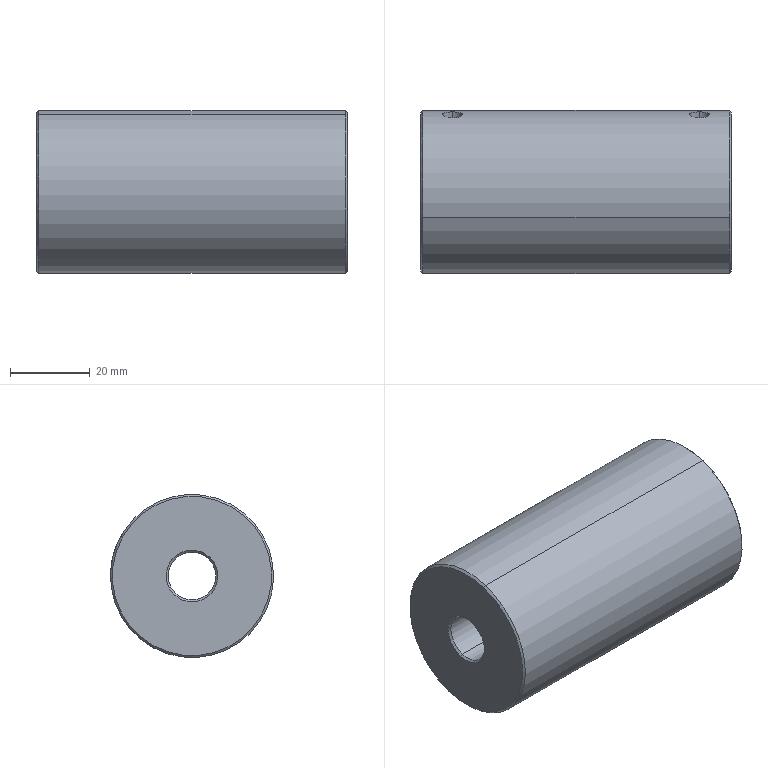Component | SolidWorks | ConveyorDriveWheel-1 | 1 solid | 18 faces | box 78 x 41 x 41 mm | volume 93543 mm3 | cone 8 | cylinder 8 | plane 2 | commonest cylinder face diameters 5 x4 12 x2 41 x2 | material Plain Carbon Steel
build123d program:
from build123d import *

# Parameters (mm, degrees)
SKETCH3_R             = 20.5
BOSS_EXTRUDE1_DEPTH   = 78
SKETCH6_R             = 6
CUT_EXTRUDE2_DEPTH    = 84.214
M6_TAPPED_HOLE1_D     = 5
M6_TAPPED_HOLE1_DEPTH = 22
M6_TAPPED_HOLE1_TIP   = 1.502
CHAMFER1_SIZE         = 0.5


with BuildPart() as part:
    # Sketch3 → Boss-Extrude1 (new body)
    with BuildSketch(Plane(origin=(0, 0, 0), x_dir=(0, 0, -1), z_dir=(1, 0, 0))):
        Circle(SKETCH3_R)
    extrude(amount=BOSS_EXTRUDE1_DEPTH)

    # Sketch6 → Cut-Extrude2 (cut, through all)
    with BuildSketch(Plane.ZY):
        Circle(SKETCH6_R)
    extrude(amount=-CUT_EXTRUDE2_DEPTH, mode=Mode.SUBTRACT)

    # M6 Tapped Hole1
    with Locations(Plane(origin=(0, 20.5, 0), x_dir=(1, 0, 0), z_dir=(0, 1, 0))):
        with Locations((8, 0), (70, 0)):
            Hole(M6_TAPPED_HOLE1_D / 2, depth=M6_TAPPED_HOLE1_DEPTH)
            with Locations((0, 0, -(M6_TAPPED_HOLE1_DEPTH + M6_TAPPED_HOLE1_TIP / 2))):  # 118° drill point
                Cone(0, M6_TAPPED_HOLE1_D / 2, M6_TAPPED_HOLE1_TIP, mode=Mode.SUBTRACT)

    # Chamfer1
    chamfer1_edges = [part.edges().sort_by_distance(p)[0] for p in [
        (0, 0, 20.5),
        (78, 0, 20.5),
        (78, 0, -6),
        (0, 0, -6),
    ]]
    chamfer(chamfer1_edges, length=CHAMFER1_SIZE)


solid = part.part

# Placed as in the assembly
solid = solid.moved(Location((-43.55, 5.646, 1535), (18.125, 0, 0)))
STEP:
#1=COLOUR_RGB('',0.7922,0.8196,0.9333);
#2=FILL_AREA_STYLE_COLOUR('',#1);
#3=FILL_AREA_STYLE('',(#2));
#4=SURFACE_STYLE_FILL_AREA(#3);
#5=SURFACE_SIDE_STYLE('',(#4));
#6=SURFACE_STYLE_USAGE(.BOTH.,#5);
#7=PRESENTATION_STYLE_ASSIGNMENT((#6));
#8=CARTESIAN_POINT('',(1.356,0.4671,59.685));
#9=VERTEX_POINT('',#8);
#10=CARTESIAN_POINT('',(1.356,-0.0226,61.181));
#11=VERTEX_POINT('',#10);
#12=CARTESIAN_POINT('',(1.356,0.2223,60.433));
#13=DIRECTION('',(1.,0.,0.));
#14=DIRECTION('',(0.,0.311,-0.9504));
#15=AXIS2_PLACEMENT_3D('',#12,#13,#14);
#16=CIRCLE('',#15,0.7874);
#17=EDGE_CURVE('',#9,#11,#16,.T.);
#18=ORIENTED_EDGE('',*,*,#17,.F.);
#19=CARTESIAN_POINT('',(1.337,0.4733,59.666));
#20=VERTEX_POINT('',#19);
#21=CARTESIAN_POINT('',(1.356,0.4671,59.685));
#22=DIRECTION('',(-0.7071,0.2199,-0.672));
#23=VECTOR('',#22,39.37);
#24=LINE('',#21,#23);
#25=EDGE_CURVE('',#9,#20,#24,.T.);
#26=ORIENTED_EDGE('',*,*,#25,.T.);
#27=CARTESIAN_POINT('',(1.337,-0.02873,61.2));
#28=VERTEX_POINT('',#27);
#29=CARTESIAN_POINT('',(1.337,0.2223,60.433));
#30=DIRECTION('',(-1.,0.,0.));
#31=DIRECTION('',(0.,0.311,-0.9504));
#32=AXIS2_PLACEMENT_3D('',#29,#30,#31);
#33=CIRCLE('',#32,0.8071);
#34=EDGE_CURVE('',#28,#20,#33,.T.);
#35=ORIENTED_EDGE('',*,*,#34,.F.);
#36=CARTESIAN_POINT('',(1.356,-0.0226,61.181));
#37=DIRECTION('',(-0.7071,-0.2199,0.672));
#38=VECTOR('',#37,39.37);
#39=LINE('',#36,#38);
#40=EDGE_CURVE('',#11,#28,#39,.T.);
#41=ORIENTED_EDGE('',*,*,#40,.F.);
#42=EDGE_LOOP('',(#18,#26,#35,#41));
#43=FACE_OUTER_BOUND('',#42,.T.);
#44=CARTESIAN_POINT('',(1.356,0.2223,60.433));
#45=DIRECTION('',(-1.,0.,0.));
#46=DIRECTION('',(0.,-0.311,0.9504));
#47=AXIS2_PLACEMENT_3D('',#44,#45,#46);
#48=CONICAL_SURFACE('',#47,0.7874,0.7854);
#49=ADVANCED_FACE('',(#43),#48,.T.);
#50=CARTESIAN_POINT('',(1.337,0.1488,60.658));
#51=VERTEX_POINT('',#50);
#52=CARTESIAN_POINT('',(1.337,0.2957,60.209));
#53=VERTEX_POINT('',#52);
#54=CARTESIAN_POINT('',(1.337,0.2223,60.433));
#55=DIRECTION('',(1.,0.,0.));
#56=DIRECTION('',(0.,0.311,-0.9504));
#57=AXIS2_PLACEMENT_3D('',#54,#55,#56);
#58=CIRCLE('',#57,0.2362);
#59=EDGE_CURVE('',#51,#53,#58,.T.);
#60=ORIENTED_EDGE('',*,*,#59,.F.);
#61=CARTESIAN_POINT('',(1.356,0.1427,60.676));
#62=VERTEX_POINT('',#61);
#63=CARTESIAN_POINT('',(1.356,0.1427,60.676));
#64=DIRECTION('',(0.7071,-0.2199,0.672));
#65=VECTOR('',#64,39.37);
#66=LINE('',#63,#65);
#67=EDGE_CURVE('',#51,#62,#66,.T.);
#68=ORIENTED_EDGE('',*,*,#67,.T.);
#69=CARTESIAN_POINT('',(1.356,0.3019,60.19));
#70=VERTEX_POINT('',#69);
#71=CARTESIAN_POINT('',(1.356,0.2223,60.433));
#72=DIRECTION('',(-1.,0.,0.));
#73=DIRECTION('',(0.,0.311,-0.9504));
#74=AXIS2_PLACEMENT_3D('',#71,#72,#73);
#75=CIRCLE('',#74,0.2559);
#76=EDGE_CURVE('',#70,#62,#75,.T.);
#77=ORIENTED_EDGE('',*,*,#76,.F.);
#78=CARTESIAN_POINT('',(1.356,0.3019,60.19));
#79=DIRECTION('',(0.7071,0.2199,-0.672));
#80=VECTOR('',#79,39.37);
#81=LINE('',#78,#80);
#82=EDGE_CURVE('',#53,#70,#81,.T.);
#83=ORIENTED_EDGE('',*,*,#82,.F.);
#84=EDGE_LOOP('',(#60,#68,#77,#83));
#85=FACE_OUTER_BOUND('',#84,.T.);
#86=CARTESIAN_POINT('',(1.356,0.2223,60.433));
#87=DIRECTION('',(1.,0.,0.));
#88=DIRECTION('',(0.,0.311,-0.9504));
#89=AXIS2_PLACEMENT_3D('',#86,#87,#88);
#90=CONICAL_SURFACE('',#89,0.2559,0.7854);
#91=ADVANCED_FACE('',(#85),#90,.F.);
#92=CARTESIAN_POINT('',(-1.715,-0.0226,61.181));
#93=VERTEX_POINT('',#92);
#94=CARTESIAN_POINT('',(-1.715,0.4671,59.685));
#95=VERTEX_POINT('',#94);
#96=CARTESIAN_POINT('',(-1.715,0.2223,60.433));
#97=DIRECTION('',(-1.,0.,0.));
#98=DIRECTION('',(0.,0.311,-0.9504));
#99=AXIS2_PLACEMENT_3D('',#96,#97,#98);
#100=CIRCLE('',#99,0.7874);
#101=EDGE_CURVE('',#93,#95,#100,.T.);
#102=ORIENTED_EDGE('',*,*,#101,.F.);
#103=CARTESIAN_POINT('',(-1.695,-0.02873,61.2));
#104=VERTEX_POINT('',#103);
#105=CARTESIAN_POINT('',(-1.695,-0.02873,61.2));
#106=DIRECTION('',(0.7071,-0.2199,0.672));
#107=VECTOR('',#106,39.37);
#108=LINE('',#105,#107);
#109=EDGE_CURVE('',#93,#104,#108,.T.);
#110=ORIENTED_EDGE('',*,*,#109,.T.);
#111=CARTESIAN_POINT('',(-1.695,0.4733,59.666));
#112=VERTEX_POINT('',#111);
#113=CARTESIAN_POINT('',(-1.695,0.2223,60.433));
#114=DIRECTION('',(1.,0.,0.));
#115=DIRECTION('',(0.,0.311,-0.9504));
#116=AXIS2_PLACEMENT_3D('',#113,#114,#115);
#117=CIRCLE('',#116,0.8071);
#118=EDGE_CURVE('',#112,#104,#117,.T.);
#119=ORIENTED_EDGE('',*,*,#118,.F.);
#120=CARTESIAN_POINT('',(-1.695,0.4733,59.666));
#121=DIRECTION('',(0.7071,0.2199,-0.672));
#122=VECTOR('',#121,39.37);
#123=LINE('',#120,#122);
#124=EDGE_CURVE('',#95,#112,#123,.T.);
#125=ORIENTED_EDGE('',*,*,#124,.F.);
#126=EDGE_LOOP('',(#102,#110,#119,#125));
#127=FACE_OUTER_BOUND('',#126,.T.);
#128=CARTESIAN_POINT('',(-1.695,0.2223,60.433));
#129=DIRECTION('',(1.,0.,0.));
#130=DIRECTION('',(0.,0.311,-0.9504));
#131=AXIS2_PLACEMENT_3D('',#128,#129,#130);
#132=CONICAL_SURFACE('',#131,0.8071,0.7854);
#133=ADVANCED_FACE('',(#127),#132,.T.);
#134=CARTESIAN_POINT('',(-1.695,0.2957,60.209));
#135=VERTEX_POINT('',#134);
#136=CARTESIAN_POINT('',(-1.695,0.1488,60.658));
#137=VERTEX_POINT('',#136);
#138=CARTESIAN_POINT('',(-1.695,0.2223,60.433));
#139=DIRECTION('',(-1.,0.,0.));
#140=DIRECTION('',(0.,0.311,-0.9504));
#141=AXIS2_PLACEMENT_3D('',#138,#139,#140);
#142=CIRCLE('',#141,0.2362);
#143=EDGE_CURVE('',#135,#137,#142,.T.);
#144=ORIENTED_EDGE('',*,*,#143,.F.);
#145=CARTESIAN_POINT('',(-1.715,0.3019,60.19));
#146=VERTEX_POINT('',#145);
#147=CARTESIAN_POINT('',(-1.695,0.2957,60.209));
#148=DIRECTION('',(-0.7071,0.2199,-0.672));
#149=VECTOR('',#148,39.37);
#150=LINE('',#147,#149);
#151=EDGE_CURVE('',#135,#146,#150,.T.);
#152=ORIENTED_EDGE('',*,*,#151,.T.);
#153=CARTESIAN_POINT('',(-1.715,0.1427,60.676));
#154=VERTEX_POINT('',#153);
#155=CARTESIAN_POINT('',(-1.715,0.2223,60.433));
#156=DIRECTION('',(1.,0.,0.));
#157=DIRECTION('',(0.,0.311,-0.9504));
#158=AXIS2_PLACEMENT_3D('',#155,#156,#157);
#159=CIRCLE('',#158,0.2559);
#160=EDGE_CURVE('',#154,#146,#159,.T.);
#161=ORIENTED_EDGE('',*,*,#160,.F.);
#162=CARTESIAN_POINT('',(-1.695,0.1488,60.658));
#163=DIRECTION('',(-0.7071,-0.2199,0.672));
#164=VECTOR('',#163,39.37);
#165=LINE('',#162,#164);
#166=EDGE_CURVE('',#137,#154,#165,.T.);
#167=ORIENTED_EDGE('',*,*,#166,.F.);
#168=EDGE_LOOP('',(#144,#152,#161,#167));
#169=FACE_OUTER_BOUND('',#168,.T.);
#170=CARTESIAN_POINT('',(-1.695,0.2223,60.433));
#171=DIRECTION('',(-1.,0.,0.));
#172=DIRECTION('',(0.,-0.311,0.9504));
#173=AXIS2_PLACEMENT_3D('',#170,#171,#172);
#174=CONICAL_SURFACE('',#173,0.2362,0.7854);
#175=ADVANCED_FACE('',(#169),#174,.F.);
#176=CARTESIAN_POINT('',(-1.4,0.457,60.406));
#177=VERTEX_POINT('',#176);
#178=CARTESIAN_POINT('',(-1.4,0.3958,60.593));
#179=VERTEX_POINT('',#178);
#180=CARTESIAN_POINT('',(-1.4,0.457,60.406));
#181=CARTESIAN_POINT('',(-1.406,0.457,60.406));
#182=CARTESIAN_POINT('',(-1.413,0.4571,60.407));
#183=CARTESIAN_POINT('',(-1.425,0.4573,60.41));
#184=CARTESIAN_POINT('',(-1.432,0.4576,60.412));
#185=CARTESIAN_POINT('',(-1.443,0.458,60.417));
#186=CARTESIAN_POINT('',(-1.449,0.4582,60.421));
#187=CARTESIAN_POINT('',(-1.46,0.4585,60.428));
#188=CARTESIAN_POINT('',(-1.465,0.4585,60.432));
#189=CARTESIAN_POINT('',(-1.474,0.4584,60.442));
#190=CARTESIAN_POINT('',(-1.478,0.4581,60.447));
#191=CARTESIAN_POINT('',(-1.485,0.4573,60.458));
#192=CARTESIAN_POINT('',(-1.488,0.4566,60.464));
#193=CARTESIAN_POINT('',(-1.493,0.4547,60.476));
#194=CARTESIAN_POINT('',(-1.495,0.4535,60.482));
#195=CARTESIAN_POINT('',(-1.497,0.4506,60.494));
#196=CARTESIAN_POINT('',(-1.498,0.4488,60.5));
#197=CARTESIAN_POINT('',(-1.498,0.4427,60.519));
#198=CARTESIAN_POINT('',(-1.495,0.4376,60.531));
#199=CARTESIAN_POINT('',(-1.488,0.4293,60.547));
#200=CARTESIAN_POINT('',(-1.485,0.4264,60.552));
#201=CARTESIAN_POINT('',(-1.478,0.4207,60.561));
#202=CARTESIAN_POINT('',(-1.474,0.4179,60.566));
#203=CARTESIAN_POINT('',(-1.465,0.4124,60.573));
#204=CARTESIAN_POINT('',(-1.46,0.4098,60.577));
#205=CARTESIAN_POINT('',(-1.449,0.4051,60.583));
#206=CARTESIAN_POINT('',(-1.444,0.403,60.585));
#207=CARTESIAN_POINT('',(-1.432,0.3995,60.589));
#208=CARTESIAN_POINT('',(-1.425,0.3981,60.591));
#209=CARTESIAN_POINT('',(-1.413,0.3963,60.593));
#210=CARTESIAN_POINT('',(-1.406,0.3958,60.593));
#211=CARTESIAN_POINT('',(-1.4,0.3958,60.593));
#212=B_SPLINE_CURVE_WITH_KNOTS('',3,(#180,#181,#182,#183,#184,#185,#186,#187,#188,#189,#190,#191,#192,#193,#194,#195,#196,#197,#198,#199,#200,#201,#202,#203,#204,#205,#206,#207,#208,#209,#210,#211),.UNSPECIFIED.,.F.,.F.,(4,2,2,2,2,2,2,2,2,2,2,2,2,2,2,4),(0.007907,0.008401,0.008895,0.009388,0.009882,0.01038,0.01087,0.01136,0.01186,0.01284,0.01334,0.01383,0.01433,0.01482,0.01531,0.01581),.UNSPECIFIED.);
#213=EDGE_CURVE('',#177,#179,#212,.T.);
#214=ORIENTED_EDGE('',*,*,#213,.F.);
#215=CARTESIAN_POINT('',(-1.4,1.014,60.589));
#216=VERTEX_POINT('',#215);
#217=CARTESIAN_POINT('',(-1.4,1.02,60.591));
#218=DIRECTION('',(0.,0.9504,0.311));
#219=VECTOR('',#218,39.37);
#220=LINE('',#217,#219);
#221=EDGE_CURVE('',#177,#216,#220,.T.);
#222=ORIENTED_EDGE('',*,*,#221,.T.);
#223=CARTESIAN_POINT('',(-1.4,0.953,60.776));
#224=VERTEX_POINT('',#223);
#225=CARTESIAN_POINT('',(-1.4,0.953,60.776));
#226=CARTESIAN_POINT('',(-1.406,0.953,60.776));
#227=CARTESIAN_POINT('',(-1.412,0.9533,60.775));
#228=CARTESIAN_POINT('',(-1.425,0.9543,60.773));
#229=CARTESIAN_POINT('',(-1.431,0.9551,60.771));
#230=CARTESIAN_POINT('',(-1.443,0.9572,60.767));
#231=CARTESIAN_POINT('',(-1.449,0.9585,60.764));
#232=CARTESIAN_POINT('',(-1.46,0.9614,60.757));
#233=CARTESIAN_POINT('',(-1.465,0.9631,60.753));
#234=CARTESIAN_POINT('',(-1.474,0.9666,60.745));
#235=CARTESIAN_POINT('',(-1.478,0.9685,60.74));
#236=CARTESIAN_POINT('',(-1.485,0.9726,60.73));
#237=CARTESIAN_POINT('',(-1.488,0.9747,60.725));
#238=CARTESIAN_POINT('',(-1.493,0.9789,60.714));
#239=CARTESIAN_POINT('',(-1.495,0.981,60.708));
#240=CARTESIAN_POINT('',(-1.497,0.9853,60.696));
#241=CARTESIAN_POINT('',(-1.498,0.9873,60.69));
#242=CARTESIAN_POINT('',(-1.498,0.9913,60.678));
#243=CARTESIAN_POINT('',(-1.497,0.9933,60.672));
#244=CARTESIAN_POINT('',(-1.495,0.9969,60.66));
#245=CARTESIAN_POINT('',(-1.493,0.9986,60.654));
#246=CARTESIAN_POINT('',(-1.488,1.002,60.642));
#247=CARTESIAN_POINT('',(-1.485,1.003,60.637));
#248=CARTESIAN_POINT('',(-1.478,1.006,60.626));
#249=CARTESIAN_POINT('',(-1.474,1.007,60.621));
#250=CARTESIAN_POINT('',(-1.465,1.009,60.613));
#251=CARTESIAN_POINT('',(-1.46,1.01,60.609));
#252=CARTESIAN_POINT('',(-1.449,1.012,60.602));
#253=CARTESIAN_POINT('',(-1.443,1.012,60.598));
#254=CARTESIAN_POINT('',(-1.431,1.013,60.594));
#255=CARTESIAN_POINT('',(-1.425,1.014,60.592));
#256=CARTESIAN_POINT('',(-1.413,1.014,60.589));
#257=CARTESIAN_POINT('',(-1.406,1.014,60.589));
#258=CARTESIAN_POINT('',(-1.4,1.014,60.589));
#259=B_SPLINE_CURVE_WITH_KNOTS('',3,(#225,#226,#227,#228,#229,#230,#231,#232,#233,#234,#235,#236,#237,#238,#239,#240,#241,#242,#243,#244,#245,#246,#247,#248,#249,#250,#251,#252,#253,#254,#255,#256,#257,#258),.UNSPECIFIED.,.F.,.F.,(4,2,2,2,2,2,2,2,2,2,2,2,2,2,2,2,4),(0.,0.000489,0.0009779,0.001467,0.001956,0.002445,0.002934,0.003423,0.003912,0.004401,0.00489,0.005379,0.005868,0.006357,0.006845,0.007334,0.007823),.UNSPECIFIED.);
#260=EDGE_CURVE('',#224,#216,#259,.T.);
#261=ORIENTED_EDGE('',*,*,#260,.F.);
#262=CARTESIAN_POINT('',(-1.4,0.9587,60.778));
#263=DIRECTION('',(0.,0.9504,0.311));
#264=VECTOR('',#263,39.37);
#265=LINE('',#262,#264);
#266=EDGE_CURVE('',#179,#224,#265,.T.);
#267=ORIENTED_EDGE('',*,*,#266,.F.);
#268=EDGE_LOOP('',(#214,#222,#261,#267));
#269=FACE_OUTER_BOUND('',#268,.T.);
#270=CARTESIAN_POINT('',(-1.4,0.9893,60.684));
#271=DIRECTION('',(0.,0.9504,0.311));
#272=DIRECTION('',(0.,-0.311,0.9504));
#273=AXIS2_PLACEMENT_3D('',#270,#271,#272);
#274=CYLINDRICAL_SURFACE('',#273,0.09843);
#275=ADVANCED_FACE('',(#269),#274,.F.);
#276=CARTESIAN_POINT('',(1.041,0.457,60.406));
#277=VERTEX_POINT('',#276);
#278=CARTESIAN_POINT('',(1.041,0.3958,60.593));
#279=VERTEX_POINT('',#278);
#280=CARTESIAN_POINT('',(1.041,0.457,60.406));
#281=CARTESIAN_POINT('',(1.035,0.457,60.406));
#282=CARTESIAN_POINT('',(1.028,0.4571,60.407));
#283=CARTESIAN_POINT('',(1.016,0.4573,60.41));
#284=CARTESIAN_POINT('',(1.009,0.4576,60.412));
#285=CARTESIAN_POINT('',(0.9975,0.458,60.417));
#286=CARTESIAN_POINT('',(0.9918,0.4582,60.421));
#287=CARTESIAN_POINT('',(0.9812,0.4585,60.428));
#288=CARTESIAN_POINT('',(0.9763,0.4585,60.432));
#289=CARTESIAN_POINT('',(0.9672,0.4584,60.442));
#290=CARTESIAN_POINT('',(0.9632,0.4581,60.447));
#291=CARTESIAN_POINT('',(0.9561,0.4573,60.458));
#292=CARTESIAN_POINT('',(0.953,0.4566,60.464));
#293=CARTESIAN_POINT('',(0.948,0.4547,60.476));
#294=CARTESIAN_POINT('',(0.9462,0.4535,60.482));
#295=CARTESIAN_POINT('',(0.9436,0.4506,60.494));
#296=CARTESIAN_POINT('',(0.9429,0.4488,60.5));
#297=CARTESIAN_POINT('',(0.9429,0.4427,60.519));
#298=CARTESIAN_POINT('',(0.9456,0.4376,60.531));
#299=CARTESIAN_POINT('',(0.953,0.4293,60.547));
#300=CARTESIAN_POINT('',(0.9561,0.4264,60.552));
#301=CARTESIAN_POINT('',(0.9632,0.4207,60.561));
#302=CARTESIAN_POINT('',(0.9673,0.4179,60.566));
#303=CARTESIAN_POINT('',(0.9763,0.4124,60.573));
#304=CARTESIAN_POINT('',(0.9813,0.4098,60.577));
#305=CARTESIAN_POINT('',(0.9918,0.4051,60.583));
#306=CARTESIAN_POINT('',(0.9974,0.403,60.585));
#307=CARTESIAN_POINT('',(1.009,0.3995,60.589));
#308=CARTESIAN_POINT('',(1.016,0.3981,60.591));
#309=CARTESIAN_POINT('',(1.028,0.3963,60.593));
#310=CARTESIAN_POINT('',(1.035,0.3958,60.593));
#311=CARTESIAN_POINT('',(1.041,0.3958,60.593));
#312=B_SPLINE_CURVE_WITH_KNOTS('',3,(#280,#281,#282,#283,#284,#285,#286,#287,#288,#289,#290,#291,#292,#293,#294,#295,#296,#297,#298,#299,#300,#301,#302,#303,#304,#305,#306,#307,#308,#309,#310,#311),.UNSPECIFIED.,.F.,.F.,(4,2,2,2,2,2,2,2,2,2,2,2,2,2,2,4),(0.007907,0.008401,0.008895,0.009388,0.009882,0.01038,0.01087,0.01136,0.01186,0.01284,0.01334,0.01383,0.01433,0.01482,0.01531,0.01581),.UNSPECIFIED.);
#313=EDGE_CURVE('',#277,#279,#312,.T.);
#314=ORIENTED_EDGE('',*,*,#313,.F.);
#315=CARTESIAN_POINT('',(1.041,1.014,60.589));
#316=VERTEX_POINT('',#315);
#317=CARTESIAN_POINT('',(1.041,1.02,60.591));
#318=DIRECTION('',(0.,0.9504,0.311));
#319=VECTOR('',#318,39.37);
#320=LINE('',#317,#319);
#321=EDGE_CURVE('',#277,#316,#320,.T.);
#322=ORIENTED_EDGE('',*,*,#321,.T.);
#323=CARTESIAN_POINT('',(1.041,0.953,60.776));
#324=VERTEX_POINT('',#323);
#325=CARTESIAN_POINT('',(1.041,0.953,60.776));
#326=CARTESIAN_POINT('',(1.035,0.953,60.776));
#327=CARTESIAN_POINT('',(1.028,0.9533,60.775));
#328=CARTESIAN_POINT('',(1.016,0.9543,60.773));
#329=CARTESIAN_POINT('',(1.01,0.9551,60.771));
#330=CARTESIAN_POINT('',(0.9977,0.9572,60.767));
#331=CARTESIAN_POINT('',(0.992,0.9585,60.764));
#332=CARTESIAN_POINT('',(0.9813,0.9614,60.757));
#333=CARTESIAN_POINT('',(0.9763,0.9631,60.753));
#334=CARTESIAN_POINT('',(0.9672,0.9666,60.745));
#335=CARTESIAN_POINT('',(0.9631,0.9685,60.74));
#336=CARTESIAN_POINT('',(0.9559,0.9726,60.73));
#337=CARTESIAN_POINT('',(0.9529,0.9747,60.725));
#338=CARTESIAN_POINT('',(0.948,0.9789,60.714));
#339=CARTESIAN_POINT('',(0.9461,0.981,60.708));
#340=CARTESIAN_POINT('',(0.9436,0.9853,60.696));
#341=CARTESIAN_POINT('',(0.9429,0.9873,60.69));
#342=CARTESIAN_POINT('',(0.9429,0.9913,60.678));
#343=CARTESIAN_POINT('',(0.9436,0.9933,60.672));
#344=CARTESIAN_POINT('',(0.9461,0.9969,60.66));
#345=CARTESIAN_POINT('',(0.9479,0.9986,60.654));
#346=CARTESIAN_POINT('',(0.9529,1.002,60.642));
#347=CARTESIAN_POINT('',(0.956,1.003,60.637));
#348=CARTESIAN_POINT('',(0.9631,1.006,60.626));
#349=CARTESIAN_POINT('',(0.9672,1.007,60.621));
#350=CARTESIAN_POINT('',(0.9763,1.009,60.613));
#351=CARTESIAN_POINT('',(0.9813,1.01,60.609));
#352=CARTESIAN_POINT('',(0.992,1.012,60.602));
#353=CARTESIAN_POINT('',(0.9977,1.012,60.598));
#354=CARTESIAN_POINT('',(1.01,1.013,60.594));
#355=CARTESIAN_POINT('',(1.016,1.014,60.592));
#356=CARTESIAN_POINT('',(1.028,1.014,60.589));
#357=CARTESIAN_POINT('',(1.035,1.014,60.589));
#358=CARTESIAN_POINT('',(1.041,1.014,60.589));
#359=B_SPLINE_CURVE_WITH_KNOTS('',3,(#325,#326,#327,#328,#329,#330,#331,#332,#333,#334,#335,#336,#337,#338,#339,#340,#341,#342,#343,#344,#345,#346,#347,#348,#349,#350,#351,#352,#353,#354,#355,#356,#357,#358),.UNSPECIFIED.,.F.,.F.,(4,2,2,2,2,2,2,2,2,2,2,2,2,2,2,2,4),(0.,0.000489,0.0009779,0.001467,0.001956,0.002445,0.002934,0.003423,0.003912,0.004401,0.00489,0.005379,0.005868,0.006357,0.006845,0.007334,0.007823),.UNSPECIFIED.);
#360=EDGE_CURVE('',#324,#316,#359,.T.);
#361=ORIENTED_EDGE('',*,*,#360,.F.);
#362=CARTESIAN_POINT('',(1.041,0.9587,60.778));
#363=DIRECTION('',(0.,0.9504,0.311));
#364=VECTOR('',#363,39.37);
#365=LINE('',#362,#364);
#366=EDGE_CURVE('',#279,#324,#365,.T.);
#367=ORIENTED_EDGE('',*,*,#366,.F.);
#368=EDGE_LOOP('',(#314,#322,#361,#367));
#369=FACE_OUTER_BOUND('',#368,.T.);
#370=CARTESIAN_POINT('',(1.041,0.9893,60.684));
#371=DIRECTION('',(0.,0.9504,0.311));
#372=DIRECTION('',(0.,-0.311,0.9504));
#373=AXIS2_PLACEMENT_3D('',#370,#371,#372);
#374=CYLINDRICAL_SURFACE('',#373,0.09843);
#375=ADVANCED_FACE('',(#369),#374,.F.);
#376=ORIENTED_EDGE('',*,*,#59,.T.);
#377=CARTESIAN_POINT('',(1.356,0.2957,60.209));
#378=DIRECTION('',(-1.,0.,0.));
#379=VECTOR('',#378,39.37);
#380=LINE('',#377,#379);
#381=EDGE_CURVE('',#53,#135,#380,.T.);
#382=ORIENTED_EDGE('',*,*,#381,.T.);
#383=ORIENTED_EDGE('',*,*,#143,.T.);
#384=CARTESIAN_POINT('',(1.356,0.1488,60.658));
#385=DIRECTION('',(-1.,0.,0.));
#386=VECTOR('',#385,39.37);
#387=LINE('',#384,#386);
#388=EDGE_CURVE('',#51,#137,#387,.T.);
#389=ORIENTED_EDGE('',*,*,#388,.F.);
#390=EDGE_LOOP('',(#376,#382,#383,#389));
#391=FACE_OUTER_BOUND('',#390,.T.);
#392=CARTESIAN_POINT('',(1.356,0.2223,60.433));
#393=DIRECTION('',(-1.,0.,0.));
#394=DIRECTION('',(0.,-0.311,0.9504));
#395=AXIS2_PLACEMENT_3D('',#392,#393,#394);
#396=CYLINDRICAL_SURFACE('',#395,0.2362);
#397=ADVANCED_FACE('',(#391),#396,.F.);
#398=ORIENTED_EDGE('',*,*,#260,.T.);
#399=CARTESIAN_POINT('',(-1.4,1.014,60.589));
#400=CARTESIAN_POINT('',(-1.393,1.014,60.589));
#401=CARTESIAN_POINT('',(-1.387,1.014,60.589));
#402=CARTESIAN_POINT('',(-1.374,1.014,60.592));
#403=CARTESIAN_POINT('',(-1.368,1.013,60.594));
#404=CARTESIAN_POINT('',(-1.356,1.012,60.598));
#405=CARTESIAN_POINT('',(-1.35,1.012,60.601));
#406=CARTESIAN_POINT('',(-1.34,1.01,60.609));
#407=CARTESIAN_POINT('',(-1.335,1.009,60.613));
#408=CARTESIAN_POINT('',(-1.325,1.007,60.621));
#409=CARTESIAN_POINT('',(-1.321,1.006,60.626));
#410=CARTESIAN_POINT('',(-1.314,1.003,60.637));
#411=CARTESIAN_POINT('',(-1.311,1.002,60.642));
#412=CARTESIAN_POINT('',(-1.306,0.9987,60.654));
#413=CARTESIAN_POINT('',(-1.304,0.9969,60.66));
#414=CARTESIAN_POINT('',(-1.302,0.9933,60.672));
#415=CARTESIAN_POINT('',(-1.301,0.9914,60.678));
#416=CARTESIAN_POINT('',(-1.301,0.9873,60.69));
#417=CARTESIAN_POINT('',(-1.302,0.9853,60.696));
#418=CARTESIAN_POINT('',(-1.304,0.9811,60.708));
#419=CARTESIAN_POINT('',(-1.306,0.9789,60.714));
#420=CARTESIAN_POINT('',(-1.311,0.9747,60.725));
#421=CARTESIAN_POINT('',(-1.314,0.9726,60.73));
#422=CARTESIAN_POINT('',(-1.321,0.9686,60.74));
#423=CARTESIAN_POINT('',(-1.325,0.9666,60.745));
#424=CARTESIAN_POINT('',(-1.334,0.9631,60.753));
#425=CARTESIAN_POINT('',(-1.339,0.9614,60.757));
#426=CARTESIAN_POINT('',(-1.35,0.9585,60.764));
#427=CARTESIAN_POINT('',(-1.356,0.9572,60.767));
#428=CARTESIAN_POINT('',(-1.374,0.9541,60.773));
#429=CARTESIAN_POINT('',(-1.387,0.953,60.776));
#430=CARTESIAN_POINT('',(-1.4,0.953,60.776));
#431=B_SPLINE_CURVE_WITH_KNOTS('',3,(#399,#400,#401,#402,#403,#404,#405,#406,#407,#408,#409,#410,#411,#412,#413,#414,#415,#416,#417,#418,#419,#420,#421,#422,#423,#424,#425,#426,#427,#428,#429,#430),.UNSPECIFIED.,.F.,.F.,(4,2,2,2,2,2,2,2,2,2,2,2,2,2,2,4),(0.007823,0.008312,0.008801,0.00929,0.009779,0.01027,0.01076,0.01125,0.01173,0.01222,0.01271,0.0132,0.01369,0.01418,0.01467,0.01564),.UNSPECIFIED.);
#432=EDGE_CURVE('',#216,#224,#431,.T.);
#433=ORIENTED_EDGE('',*,*,#432,.T.);
#434=EDGE_LOOP('',(#398,#433));
#435=FACE_BOUND('',#434,.T.);
#436=ORIENTED_EDGE('',*,*,#360,.T.);
#437=CARTESIAN_POINT('',(1.041,1.014,60.589));
#438=CARTESIAN_POINT('',(1.048,1.014,60.589));
#439=CARTESIAN_POINT('',(1.054,1.014,60.589));
#440=CARTESIAN_POINT('',(1.067,1.014,60.592));
#441=CARTESIAN_POINT('',(1.073,1.013,60.594));
#442=CARTESIAN_POINT('',(1.085,1.012,60.598));
#443=CARTESIAN_POINT('',(1.091,1.012,60.601));
#444=CARTESIAN_POINT('',(1.101,1.01,60.609));
#445=CARTESIAN_POINT('',(1.106,1.009,60.613));
#446=CARTESIAN_POINT('',(1.115,1.007,60.621));
#447=CARTESIAN_POINT('',(1.12,1.006,60.626));
#448=CARTESIAN_POINT('',(1.127,1.003,60.637));
#449=CARTESIAN_POINT('',(1.13,1.002,60.642));
#450=CARTESIAN_POINT('',(1.135,0.9987,60.654));
#451=CARTESIAN_POINT('',(1.137,0.9969,60.66));
#452=CARTESIAN_POINT('',(1.139,0.9933,60.672));
#453=CARTESIAN_POINT('',(1.14,0.9914,60.678));
#454=CARTESIAN_POINT('',(1.14,0.9873,60.69));
#455=CARTESIAN_POINT('',(1.139,0.9853,60.696));
#456=CARTESIAN_POINT('',(1.137,0.9811,60.708));
#457=CARTESIAN_POINT('',(1.135,0.9789,60.714));
#458=CARTESIAN_POINT('',(1.13,0.9747,60.725));
#459=CARTESIAN_POINT('',(1.127,0.9726,60.73));
#460=CARTESIAN_POINT('',(1.12,0.9686,60.74));
#461=CARTESIAN_POINT('',(1.116,0.9666,60.745));
#462=CARTESIAN_POINT('',(1.106,0.9631,60.753));
#463=CARTESIAN_POINT('',(1.102,0.9614,60.757));
#464=CARTESIAN_POINT('',(1.091,0.9585,60.764));
#465=CARTESIAN_POINT('',(1.085,0.9572,60.767));
#466=CARTESIAN_POINT('',(1.067,0.9541,60.773));
#467=CARTESIAN_POINT('',(1.054,0.953,60.776));
#468=CARTESIAN_POINT('',(1.041,0.953,60.776));
#469=B_SPLINE_CURVE_WITH_KNOTS('',3,(#437,#438,#439,#440,#441,#442,#443,#444,#445,#446,#447,#448,#449,#450,#451,#452,#453,#454,#455,#456,#457,#458,#459,#460,#461,#462,#463,#464,#465,#466,#467,#468),.UNSPECIFIED.,.F.,.F.,(4,2,2,2,2,2,2,2,2,2,2,2,2,2,2,4),(0.007823,0.008312,0.008801,0.00929,0.009779,0.01027,0.01076,0.01125,0.01173,0.01222,0.01271,0.0132,0.01369,0.01418,0.01467,0.01564),.UNSPECIFIED.);
#470=EDGE_CURVE('',#316,#324,#469,.T.);
#471=ORIENTED_EDGE('',*,*,#470,.T.);
#472=EDGE_LOOP('',(#436,#471));
#473=FACE_BOUND('',#472,.T.);
#474=ORIENTED_EDGE('',*,*,#34,.T.);
#475=CARTESIAN_POINT('',(1.356,0.4733,59.666));
#476=DIRECTION('',(-1.,0.,0.));
#477=VECTOR('',#476,39.37);
#478=LINE('',#475,#477);
#479=EDGE_CURVE('',#20,#112,#478,.T.);
#480=ORIENTED_EDGE('',*,*,#479,.T.);
#481=ORIENTED_EDGE('',*,*,#118,.T.);
#482=CARTESIAN_POINT('',(1.356,-0.02873,61.2));
#483=DIRECTION('',(-1.,0.,0.));
#484=VECTOR('',#483,39.37);
#485=LINE('',#482,#484);
#486=EDGE_CURVE('',#28,#104,#485,.T.);
#487=ORIENTED_EDGE('',*,*,#486,.F.);
#488=EDGE_LOOP('',(#474,#480,#481,#487));
#489=FACE_OUTER_BOUND('',#488,.T.);
#490=CARTESIAN_POINT('',(1.356,0.2223,60.433));
#491=DIRECTION('',(-1.,0.,0.));
#492=DIRECTION('',(0.,-0.311,0.9504));
#493=AXIS2_PLACEMENT_3D('',#490,#491,#492);
#494=CYLINDRICAL_SURFACE('',#493,0.8071);
#495=ADVANCED_FACE('',(#435,#473,#489),#494,.T.);
#496=ORIENTED_EDGE('',*,*,#479,.F.);
#497=CARTESIAN_POINT('',(1.337,0.2223,60.433));
#498=DIRECTION('',(-1.,0.,0.));
#499=DIRECTION('',(0.,0.311,-0.9504));
#500=AXIS2_PLACEMENT_3D('',#497,#498,#499);
#501=CIRCLE('',#500,0.8071);
#502=EDGE_CURVE('',#20,#28,#501,.T.);
#503=ORIENTED_EDGE('',*,*,#502,.T.);
#504=ORIENTED_EDGE('',*,*,#486,.T.);
#505=CARTESIAN_POINT('',(-1.695,0.2223,60.433));
#506=DIRECTION('',(1.,0.,0.));
#507=DIRECTION('',(0.,0.311,-0.9504));
#508=AXIS2_PLACEMENT_3D('',#505,#506,#507);
#509=CIRCLE('',#508,0.8071);
#510=EDGE_CURVE('',#104,#112,#509,.T.);
#511=ORIENTED_EDGE('',*,*,#510,.T.);
#512=EDGE_LOOP('',(#496,#503,#504,#511));
#513=FACE_OUTER_BOUND('',#512,.T.);
#514=CARTESIAN_POINT('',(1.356,0.2223,60.433));
#515=DIRECTION('',(-1.,0.,0.));
#516=DIRECTION('',(0.,-0.311,0.9504));
#517=AXIS2_PLACEMENT_3D('',#514,#515,#516);
#518=CYLINDRICAL_SURFACE('',#517,0.8071);
#519=ADVANCED_FACE('',(#513),#518,.T.);
#520=ORIENTED_EDGE('',*,*,#76,.T.);
#521=CARTESIAN_POINT('',(1.356,0.2223,60.433));
#522=DIRECTION('',(-1.,0.,0.));
#523=DIRECTION('',(0.,0.311,-0.9504));
#524=AXIS2_PLACEMENT_3D('',#521,#522,#523);
#525=CIRCLE('',#524,0.2559);
#526=EDGE_CURVE('',#62,#70,#525,.T.);
#527=ORIENTED_EDGE('',*,*,#526,.T.);
#528=EDGE_LOOP('',(#520,#527));
#529=FACE_BOUND('',#528,.T.);
#530=CARTESIAN_POINT('',(1.356,0.2223,60.433));
#531=DIRECTION('',(1.,0.,0.));
#532=DIRECTION('',(0.,0.311,-0.9504));
#533=AXIS2_PLACEMENT_3D('',#530,#531,#532);
#534=CIRCLE('',#533,0.7874);
#535=EDGE_CURVE('',#11,#9,#534,.T.);
#536=ORIENTED_EDGE('',*,*,#535,.T.);
#537=ORIENTED_EDGE('',*,*,#17,.T.);
#538=EDGE_LOOP('',(#536,#537));
#539=FACE_OUTER_BOUND('',#538,.T.);
#540=CARTESIAN_POINT('',(1.356,0.2223,60.433));
#541=DIRECTION('',(1.,0.,0.));
#542=DIRECTION('',(0.,0.311,-0.9504));
#543=AXIS2_PLACEMENT_3D('',#540,#541,#542);
#544=PLANE('',#543);
#545=ADVANCED_FACE('',(#529,#539),#544,.T.);
#546=ORIENTED_EDGE('',*,*,#160,.T.);
#547=CARTESIAN_POINT('',(-1.715,0.2223,60.433));
#548=DIRECTION('',(1.,0.,0.));
#549=DIRECTION('',(0.,0.311,-0.9504));
#550=AXIS2_PLACEMENT_3D('',#547,#548,#549);
#551=CIRCLE('',#550,0.2559);
#552=EDGE_CURVE('',#146,#154,#551,.T.);
#553=ORIENTED_EDGE('',*,*,#552,.T.);
#554=EDGE_LOOP('',(#546,#553));
#555=FACE_BOUND('',#554,.T.);
#556=CARTESIAN_POINT('',(-1.715,0.2223,60.433));
#557=DIRECTION('',(-1.,0.,0.));
#558=DIRECTION('',(0.,0.311,-0.9504));
#559=AXIS2_PLACEMENT_3D('',#556,#557,#558);
#560=CIRCLE('',#559,0.7874);
#561=EDGE_CURVE('',#95,#93,#560,.T.);
#562=ORIENTED_EDGE('',*,*,#561,.T.);
#563=ORIENTED_EDGE('',*,*,#101,.T.);
#564=EDGE_LOOP('',(#562,#563));
#565=FACE_OUTER_BOUND('',#564,.T.);
#566=CARTESIAN_POINT('',(-1.715,0.2223,60.433));
#567=DIRECTION('',(1.,0.,0.));
#568=DIRECTION('',(0.,0.311,-0.9504));
#569=AXIS2_PLACEMENT_3D('',#566,#567,#568);
#570=PLANE('',#569);
#571=ADVANCED_FACE('',(#555,#565),#570,.F.);
#572=ORIENTED_EDGE('',*,*,#381,.F.);
#573=CARTESIAN_POINT('',(1.337,0.2223,60.433));
#574=DIRECTION('',(1.,0.,0.));
#575=DIRECTION('',(0.,0.311,-0.9504));
#576=AXIS2_PLACEMENT_3D('',#573,#574,#575);
#577=CIRCLE('',#576,0.2362);
#578=EDGE_CURVE('',#53,#51,#577,.T.);
#579=ORIENTED_EDGE('',*,*,#578,.T.);
#580=ORIENTED_EDGE('',*,*,#388,.T.);
#581=CARTESIAN_POINT('',(-1.695,0.2223,60.433));
#582=DIRECTION('',(-1.,0.,0.));
#583=DIRECTION('',(0.,0.311,-0.9504));
#584=AXIS2_PLACEMENT_3D('',#581,#582,#583);
#585=CIRCLE('',#584,0.2362);
#586=EDGE_CURVE('',#137,#135,#585,.T.);
#587=ORIENTED_EDGE('',*,*,#586,.T.);
#588=EDGE_LOOP('',(#572,#579,#580,#587));
#589=FACE_OUTER_BOUND('',#588,.T.);
#590=CARTESIAN_POINT('',(-1.4,0.3958,60.593));
#591=CARTESIAN_POINT('',(-1.393,0.3958,60.593));
#592=CARTESIAN_POINT('',(-1.387,0.3962,60.593));
#593=CARTESIAN_POINT('',(-1.374,0.3981,60.591));
#594=CARTESIAN_POINT('',(-1.368,0.3995,60.589));
#595=CARTESIAN_POINT('',(-1.356,0.403,60.585));
#596=CARTESIAN_POINT('',(-1.35,0.4051,60.583));
#597=CARTESIAN_POINT('',(-1.339,0.4098,60.577));
#598=CARTESIAN_POINT('',(-1.334,0.4125,60.573));
#599=CARTESIAN_POINT('',(-1.321,0.4206,60.562));
#600=CARTESIAN_POINT('',(-1.314,0.4266,60.552));
#601=CARTESIAN_POINT('',(-1.306,0.4348,60.536));
#602=CARTESIAN_POINT('',(-1.304,0.4375,60.531));
#603=CARTESIAN_POINT('',(-1.302,0.4425,60.519));
#604=CARTESIAN_POINT('',(-1.301,0.4447,60.513));
#605=CARTESIAN_POINT('',(-1.301,0.4488,60.5));
#606=CARTESIAN_POINT('',(-1.302,0.4506,60.494));
#607=CARTESIAN_POINT('',(-1.304,0.4535,60.482));
#608=CARTESIAN_POINT('',(-1.306,0.4547,60.476));
#609=CARTESIAN_POINT('',(-1.311,0.4566,60.464));
#610=CARTESIAN_POINT('',(-1.314,0.4573,60.458));
#611=CARTESIAN_POINT('',(-1.321,0.4581,60.447));
#612=CARTESIAN_POINT('',(-1.326,0.4584,60.442));
#613=CARTESIAN_POINT('',(-1.335,0.4585,60.432));
#614=CARTESIAN_POINT('',(-1.339,0.4585,60.428));
#615=CARTESIAN_POINT('',(-1.35,0.4582,60.42));
#616=CARTESIAN_POINT('',(-1.356,0.458,60.417));
#617=CARTESIAN_POINT('',(-1.368,0.4576,60.412));
#618=CARTESIAN_POINT('',(-1.374,0.4573,60.41));
#619=CARTESIAN_POINT('',(-1.387,0.4571,60.407));
#620=CARTESIAN_POINT('',(-1.393,0.457,60.406));
#621=CARTESIAN_POINT('',(-1.4,0.457,60.406));
#622=B_SPLINE_CURVE_WITH_KNOTS('',3,(#590,#591,#592,#593,#594,#595,#596,#597,#598,#599,#600,#601,#602,#603,#604,#605,#606,#607,#608,#609,#610,#611,#612,#613,#614,#615,#616,#617,#618,#619,#620,#621),.UNSPECIFIED.,.F.,.F.,(4,2,2,2,2,2,2,2,2,2,2,2,2,2,2,4),(0.,0.0004942,0.0009884,0.001483,0.001977,0.002965,0.003459,0.003953,0.004448,0.004942,0.005436,0.00593,0.006424,0.006919,0.007413,0.007907),.UNSPECIFIED.);
#623=EDGE_CURVE('',#179,#177,#622,.T.);
#624=ORIENTED_EDGE('',*,*,#623,.T.);
#625=ORIENTED_EDGE('',*,*,#213,.T.);
#626=EDGE_LOOP('',(#624,#625));
#627=FACE_BOUND('',#626,.T.);
#628=CARTESIAN_POINT('',(1.041,0.3958,60.593));
#629=CARTESIAN_POINT('',(1.048,0.3958,60.593));
#630=CARTESIAN_POINT('',(1.054,0.3962,60.593));
#631=CARTESIAN_POINT('',(1.067,0.3981,60.591));
#632=CARTESIAN_POINT('',(1.073,0.3995,60.589));
#633=CARTESIAN_POINT('',(1.085,0.403,60.585));
#634=CARTESIAN_POINT('',(1.091,0.4051,60.583));
#635=CARTESIAN_POINT('',(1.102,0.4098,60.577));
#636=CARTESIAN_POINT('',(1.106,0.4125,60.573));
#637=CARTESIAN_POINT('',(1.12,0.4206,60.562));
#638=CARTESIAN_POINT('',(1.127,0.4266,60.552));
#639=CARTESIAN_POINT('',(1.135,0.4348,60.536));
#640=CARTESIAN_POINT('',(1.137,0.4375,60.531));
#641=CARTESIAN_POINT('',(1.139,0.4425,60.519));
#642=CARTESIAN_POINT('',(1.14,0.4447,60.513));
#643=CARTESIAN_POINT('',(1.14,0.4488,60.5));
#644=CARTESIAN_POINT('',(1.139,0.4506,60.494));
#645=CARTESIAN_POINT('',(1.137,0.4535,60.482));
#646=CARTESIAN_POINT('',(1.135,0.4547,60.476));
#647=CARTESIAN_POINT('',(1.13,0.4566,60.464));
#648=CARTESIAN_POINT('',(1.127,0.4573,60.458));
#649=CARTESIAN_POINT('',(1.12,0.4581,60.447));
#650=CARTESIAN_POINT('',(1.115,0.4584,60.442));
#651=CARTESIAN_POINT('',(1.106,0.4585,60.432));
#652=CARTESIAN_POINT('',(1.101,0.4585,60.428));
#653=CARTESIAN_POINT('',(1.091,0.4582,60.42));
#654=CARTESIAN_POINT('',(1.085,0.458,60.417));
#655=CARTESIAN_POINT('',(1.073,0.4576,60.412));
#656=CARTESIAN_POINT('',(1.067,0.4573,60.41));
#657=CARTESIAN_POINT('',(1.054,0.4571,60.407));
#658=CARTESIAN_POINT('',(1.048,0.457,60.406));
#659=CARTESIAN_POINT('',(1.041,0.457,60.406));
#660=B_SPLINE_CURVE_WITH_KNOTS('',3,(#628,#629,#630,#631,#632,#633,#634,#635,#636,#637,#638,#639,#640,#641,#642,#643,#644,#645,#646,#647,#648,#649,#650,#651,#652,#653,#654,#655,#656,#657,#658,#659),.UNSPECIFIED.,.F.,.F.,(4,2,2,2,2,2,2,2,2,2,2,2,2,2,2,4),(0.,0.0004942,0.0009884,0.001483,0.001977,0.002965,0.003459,0.003953,0.004448,0.004942,0.005436,0.00593,0.006424,0.006919,0.007413,0.007907),.UNSPECIFIED.);
#661=EDGE_CURVE('',#279,#277,#660,.T.);
#662=ORIENTED_EDGE('',*,*,#661,.T.);
#663=ORIENTED_EDGE('',*,*,#313,.T.);
#664=EDGE_LOOP('',(#662,#663));
#665=FACE_BOUND('',#664,.T.);
#666=CARTESIAN_POINT('',(1.356,0.2223,60.433));
#667=DIRECTION('',(-1.,0.,0.));
#668=DIRECTION('',(0.,-0.311,0.9504));
#669=AXIS2_PLACEMENT_3D('',#666,#667,#668);
#670=CYLINDRICAL_SURFACE('',#669,0.2362);
#671=ADVANCED_FACE('',(#589,#627,#665),#670,.F.);
#672=ORIENTED_EDGE('',*,*,#321,.F.);
#673=ORIENTED_EDGE('',*,*,#661,.F.);
#674=ORIENTED_EDGE('',*,*,#366,.T.);
#675=ORIENTED_EDGE('',*,*,#470,.F.);
#676=EDGE_LOOP('',(#672,#673,#674,#675));
#677=FACE_OUTER_BOUND('',#676,.T.);
#678=CARTESIAN_POINT('',(1.041,0.9893,60.684));
#679=DIRECTION('',(0.,0.9504,0.311));
#680=DIRECTION('',(0.,-0.311,0.9504));
#681=AXIS2_PLACEMENT_3D('',#678,#679,#680);
#682=CYLINDRICAL_SURFACE('',#681,0.09843);
#683=ADVANCED_FACE('',(#677),#682,.F.);
#684=ORIENTED_EDGE('',*,*,#221,.F.);
#685=ORIENTED_EDGE('',*,*,#623,.F.);
#686=ORIENTED_EDGE('',*,*,#266,.T.);
#687=ORIENTED_EDGE('',*,*,#432,.F.);
#688=EDGE_LOOP('',(#684,#685,#686,#687));
#689=FACE_OUTER_BOUND('',#688,.T.);
#690=CARTESIAN_POINT('',(-1.4,0.9893,60.684));
#691=DIRECTION('',(0.,0.9504,0.311));
#692=DIRECTION('',(0.,-0.311,0.9504));
#693=AXIS2_PLACEMENT_3D('',#690,#691,#692);
#694=CYLINDRICAL_SURFACE('',#693,0.09843);
#695=ADVANCED_FACE('',(#689),#694,.F.);
#696=ORIENTED_EDGE('',*,*,#151,.F.);
#697=ORIENTED_EDGE('',*,*,#586,.F.);
#698=ORIENTED_EDGE('',*,*,#166,.T.);
#699=ORIENTED_EDGE('',*,*,#552,.F.);
#700=EDGE_LOOP('',(#696,#697,#698,#699));
#701=FACE_OUTER_BOUND('',#700,.T.);
#702=CARTESIAN_POINT('',(-1.695,0.2223,60.433));
#703=DIRECTION('',(-1.,0.,0.));
#704=DIRECTION('',(0.,-0.311,0.9504));
#705=AXIS2_PLACEMENT_3D('',#702,#703,#704);
#706=CONICAL_SURFACE('',#705,0.2362,0.7854);
#707=ADVANCED_FACE('',(#701),#706,.F.);
#708=ORIENTED_EDGE('',*,*,#109,.F.);
#709=ORIENTED_EDGE('',*,*,#561,.F.);
#710=ORIENTED_EDGE('',*,*,#124,.T.);
#711=ORIENTED_EDGE('',*,*,#510,.F.);
#712=EDGE_LOOP('',(#708,#709,#710,#711));
#713=FACE_OUTER_BOUND('',#712,.T.);
#714=CARTESIAN_POINT('',(-1.695,0.2223,60.433));
#715=DIRECTION('',(1.,0.,0.));
#716=DIRECTION('',(0.,0.311,-0.9504));
#717=AXIS2_PLACEMENT_3D('',#714,#715,#716);
#718=CONICAL_SURFACE('',#717,0.8071,0.7854);
#719=ADVANCED_FACE('',(#713),#718,.T.);
#720=ORIENTED_EDGE('',*,*,#67,.F.);
#721=ORIENTED_EDGE('',*,*,#578,.F.);
#722=ORIENTED_EDGE('',*,*,#82,.T.);
#723=ORIENTED_EDGE('',*,*,#526,.F.);
#724=EDGE_LOOP('',(#720,#721,#722,#723));
#725=FACE_OUTER_BOUND('',#724,.T.);
#726=CARTESIAN_POINT('',(1.356,0.2223,60.433));
#727=DIRECTION('',(1.,0.,0.));
#728=DIRECTION('',(0.,0.311,-0.9504));
#729=AXIS2_PLACEMENT_3D('',#726,#727,#728);
#730=CONICAL_SURFACE('',#729,0.2559,0.7854);
#731=ADVANCED_FACE('',(#725),#730,.F.);
#732=ORIENTED_EDGE('',*,*,#25,.F.);
#733=ORIENTED_EDGE('',*,*,#535,.F.);
#734=ORIENTED_EDGE('',*,*,#40,.T.);
#735=ORIENTED_EDGE('',*,*,#502,.F.);
#736=EDGE_LOOP('',(#732,#733,#734,#735));
#737=FACE_OUTER_BOUND('',#736,.T.);
#738=CARTESIAN_POINT('',(1.356,0.2223,60.433));
#739=DIRECTION('',(-1.,0.,0.));
#740=DIRECTION('',(0.,-0.311,0.9504));
#741=AXIS2_PLACEMENT_3D('',#738,#739,#740);
#742=CONICAL_SURFACE('',#741,0.7874,0.7854);
#743=ADVANCED_FACE('',(#737),#742,.T.);
#744=CLOSED_SHELL('',(#49,#91,#133,#175,#275,#375,#397,#495,#519,#545,#571,#671,#683,#695,#707,#719,#731,#743));
#745=MANIFOLD_SOLID_BREP('',#744);
#746=STYLED_ITEM('',(#7),#745);
#747=PRESENTATION_LAYER_ASSIGNMENT('','',(#746));
#748=(LENGTH_UNIT()NAMED_UNIT(*)SI_UNIT($,.METRE.));
#749=LENGTH_MEASURE_WITH_UNIT(LENGTH_MEASURE(0.0254),#748);
#750=DIMENSIONAL_EXPONENTS(1.,0.,0.,0.,0.,0.,0.);
#751=(CONVERSION_BASED_UNIT('',#749)LENGTH_UNIT()NAMED_UNIT(#750));
#752=UNCERTAINTY_MEASURE_WITH_UNIT(LENGTH_MEASURE(0.00001),#751,'','');
#753=(NAMED_UNIT(*)PLANE_ANGLE_UNIT()SI_UNIT($,.RADIAN.));
#754=(NAMED_UNIT(*)SI_UNIT($,.STERADIAN.)SOLID_ANGLE_UNIT());
#755=(GEOMETRIC_REPRESENTATION_CONTEXT(3)GLOBAL_UNCERTAINTY_ASSIGNED_CONTEXT((#752))GLOBAL_UNIT_ASSIGNED_CONTEXT((#751,#753,#754))REPRESENTATION_CONTEXT('',''));
#756=MECHANICAL_DESIGN_GEOMETRIC_PRESENTATION_REPRESENTATION('',(#746),#755);
#757=CARTESIAN_POINT('',(0.,0.,0.));
#758=DIRECTION('',(0.,0.,1.));
#759=DIRECTION('',(1.,0.,0.));
#760=AXIS2_PLACEMENT_3D('',#757,#758,#759);
#761=(LENGTH_UNIT()NAMED_UNIT(*)SI_UNIT($,.METRE.));
#762=LENGTH_MEASURE_WITH_UNIT(LENGTH_MEASURE(0.0254),#761);
#763=DIMENSIONAL_EXPONENTS(1.,0.,0.,0.,0.,0.,0.);
#764=(CONVERSION_BASED_UNIT('',#762)LENGTH_UNIT()NAMED_UNIT(#763));
#765=UNCERTAINTY_MEASURE_WITH_UNIT(LENGTH_MEASURE(0.00001),#764,'','');
#766=(NAMED_UNIT(*)PLANE_ANGLE_UNIT()SI_UNIT($,.RADIAN.));
#767=(NAMED_UNIT(*)SI_UNIT($,.STERADIAN.)SOLID_ANGLE_UNIT());
#768=(GEOMETRIC_REPRESENTATION_CONTEXT(3)GLOBAL_UNCERTAINTY_ASSIGNED_CONTEXT((#765))GLOBAL_UNIT_ASSIGNED_CONTEXT((#764,#766,#767))REPRESENTATION_CONTEXT('',''));
#769=ADVANCED_BREP_SHAPE_REPRESENTATION('',(#745,#760),#768);